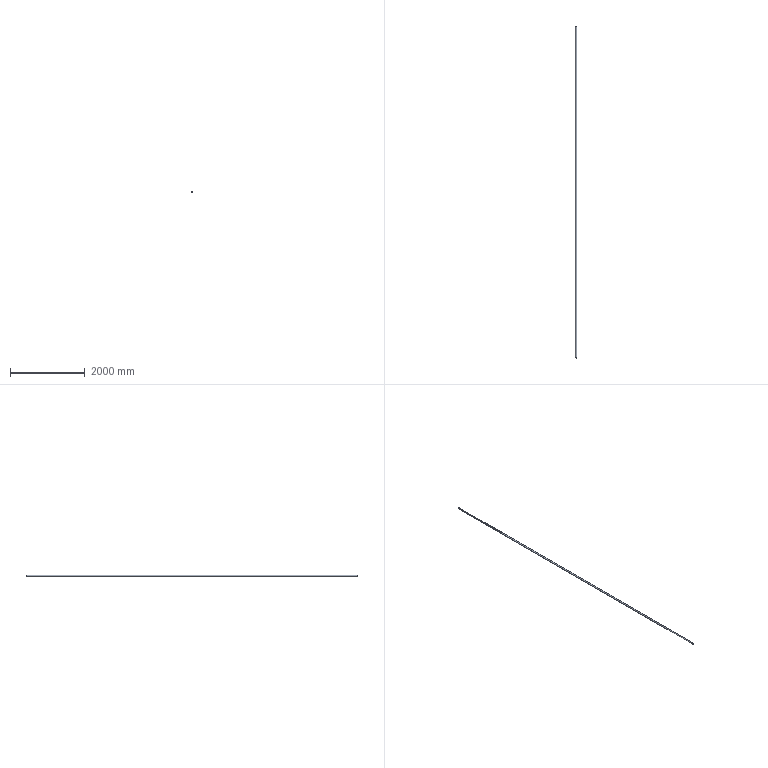Component | NX | 43_6 | 1 solid | 4 faces | volume 2979383 mm3 | cylinder 2 | plane 2 | commonest cylinder face diameters 34 x1 27 x1